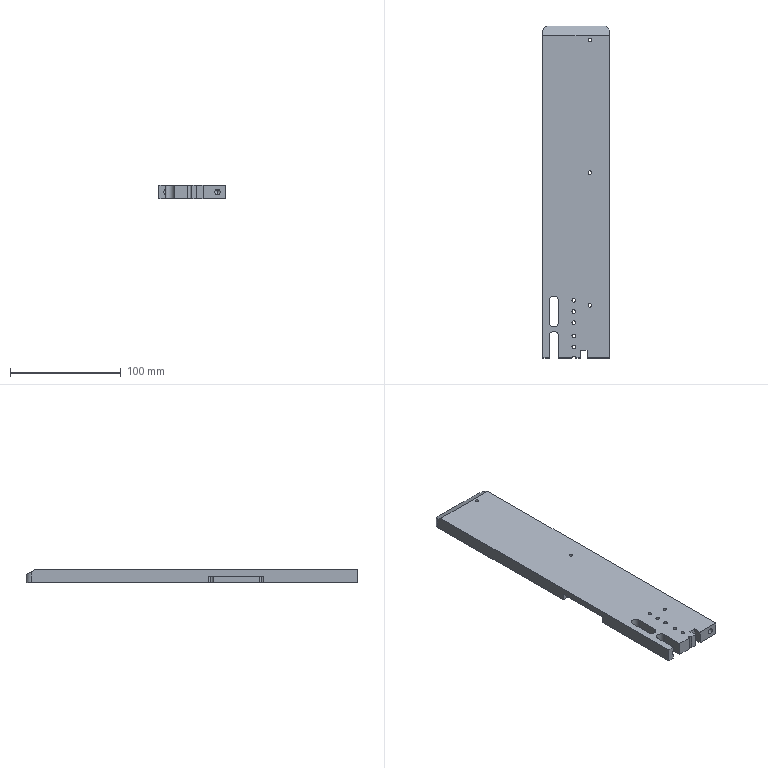Component | SolidWorks | 03-1111-2 | 1 solid | 53 faces | box 60 x 300 x 12 mm | volume 202042 mm3 | cylinder 29 | plane 21 | cone 3 | commonest cylinder face diameters 3.3 x17 4 x4 5 x3 8 x3 10 x2
build123d program:
from build123d import *

# Parameters (mm, degrees)
SKETCH1_W             = 60
SKETCH1_H             = 12
BOSS_EXTRUDE1_DEPTH   = 300
SKETCH2_W             = 20
SKETCH2_H             = 50
CUT_EXTRUDE1_DEPTH    = 6
CUT_EXTRUDE2_DEPTH    = 302.735
CHAMFER1_SIZE         = 5
CHAMFER1_SIZE2        = 8.66
FILLET1_R             = 5
SKETCH6_R             = 2
CUT_EXTRUDE3_DEPTH    = 6
M6_TAPPED_HOLE1_D     = 5
M6_TAPPED_HOLE1_DEPTH = 15
M6_TAPPED_HOLE1_TIP   = 1.502
SKETCH10_W            = 6
SKETCH10_H            = 14
CUT_EXTRUDE4_DEPTH    = 302.735
M4_TAPPED_HOLE1_D     = 3.3
LPATTERN1_COUNT       = 2
LPATTERN1_PITCH       = 32
M4_TAPPED_HOLE2_D     = 3.3


with BuildPart() as part:
    # Sketch1 → Boss-Extrude1 (new body)
    with BuildSketch(Plane(origin=(0, 0, 0), x_dir=(1, 0, 0), z_dir=(0, 1, 0))):
        Rectangle(SKETCH1_W, SKETCH1_H)
    extrude(amount=BOSS_EXTRUDE1_DEPTH)

    # Sketch2 → Cut-Extrude1 (cut)
    with BuildSketch(Plane.XY.offset(6)):
        with Locations((-20, 190)):
            Rectangle(SKETCH2_W, SKETCH2_H)
    extrude(amount=-CUT_EXTRUDE1_DEPTH, mode=Mode.SUBTRACT)

    # Sketch3 → Cut-Extrude2 (cut, through all)
    with BuildSketch(Plane.XY.offset(6)):
        with BuildLine():
            Line((-24, 280), (-24, 300))
            ThreePointArc((-24, 300), (-20, 304), (-16, 300))
            Line((-16, 300), (-16, 280))
            ThreePointArc((-16, 280), (-20, 276), (-24, 280))
        make_face()
    cut_extrude2 = extrude(amount=-CUT_EXTRUDE2_DEPTH, mode=Mode.SUBTRACT)

    # Chamfer1
    chamfer1_edges = [part.edges().sort_by_distance(p)[0] for p in [
        (0, 0, -6),
    ]]
    chamfer1_side = [part.faces().sort_by_distance(p)[0] for p in [
        (0, 0, 0),
    ]]
    chamfer(chamfer1_edges, length=CHAMFER1_SIZE, length2=CHAMFER1_SIZE2, reference=chamfer1_side[0])

    # Fillet1
    fillet1_edges = [part.edges().sort_by_distance(p)[0] for p in [
        (-30, 0, 2.5),
        (30, 0, 2.5),
    ]]
    fillet(fillet1_edges, radius=FILLET1_R)

    # Sketch6 → Cut-Extrude3 (cut)
    with BuildSketch(Plane.XY.offset(6)):
        with Locations((-10, 167)):
            Circle(SKETCH6_R)
        with Locations((-10, 213)):
            Circle(SKETCH6_R)
    extrude(amount=-CUT_EXTRUDE3_DEPTH, mode=Mode.SUBTRACT)

    # M6 Tapped Hole1
    with Locations(Plane(origin=(0, 300, 0), x_dir=(1, 0, 0), z_dir=(0, 1, 0))):
        with Locations((-23, 0), (23, 0)):
            Hole(M6_TAPPED_HOLE1_D / 2, depth=M6_TAPPED_HOLE1_DEPTH)
            with Locations((0, 0, -(M6_TAPPED_HOLE1_DEPTH + M6_TAPPED_HOLE1_TIP / 2))):  # 118° drill point
                Cone(0, M6_TAPPED_HOLE1_D / 2, M6_TAPPED_HOLE1_TIP, mode=Mode.SUBTRACT)

    # Sketch10 → Cut-Extrude4 (cut, through all)
    with BuildSketch(Plane(origin=(0, 0, -6), x_dir=(-1, 0, 0), z_dir=(0, 0, -1))):
        with Locations((-7, 300)):
            Rectangle(SKETCH10_W, SKETCH10_H)
    extrude(amount=-CUT_EXTRUDE4_DEPTH, mode=Mode.SUBTRACT)

    # M4 Tapped Hole1 (through all)
    with Locations(Plane.XY.offset(6)):
        with Locations((-2, 280), (-2, 300), (-2, 290)):
            m4_tapped_hole1 = Hole(M4_TAPPED_HOLE1_D / 2)

    # LPattern1: Cut-Extrude2, M4 Tapped Hole1 ×2
    with Locations(*[(0, -i * LPATTERN1_PITCH, 0) for i in range(1, LPATTERN1_COUNT)]):
        add(cut_extrude2, mode=Mode.SUBTRACT)
        add(m4_tapped_hole1, mode=Mode.SUBTRACT)

    # M4 Tapped Hole2 (through all)
    with Locations(Plane(origin=(0, 0, -6), x_dir=(-1, 0, 0), z_dir=(0, 0, -1))):
        with Locations((-12.5, 252.5), (-12.5, 132.5), (-12.5, 12.5)):
            Hole(M4_TAPPED_HOLE2_D / 2)


solid = part.part

# Placed as in the assembly
solid = solid.moved(Location((141.928, 706.224, 1276.056), (180, 0, 0)))